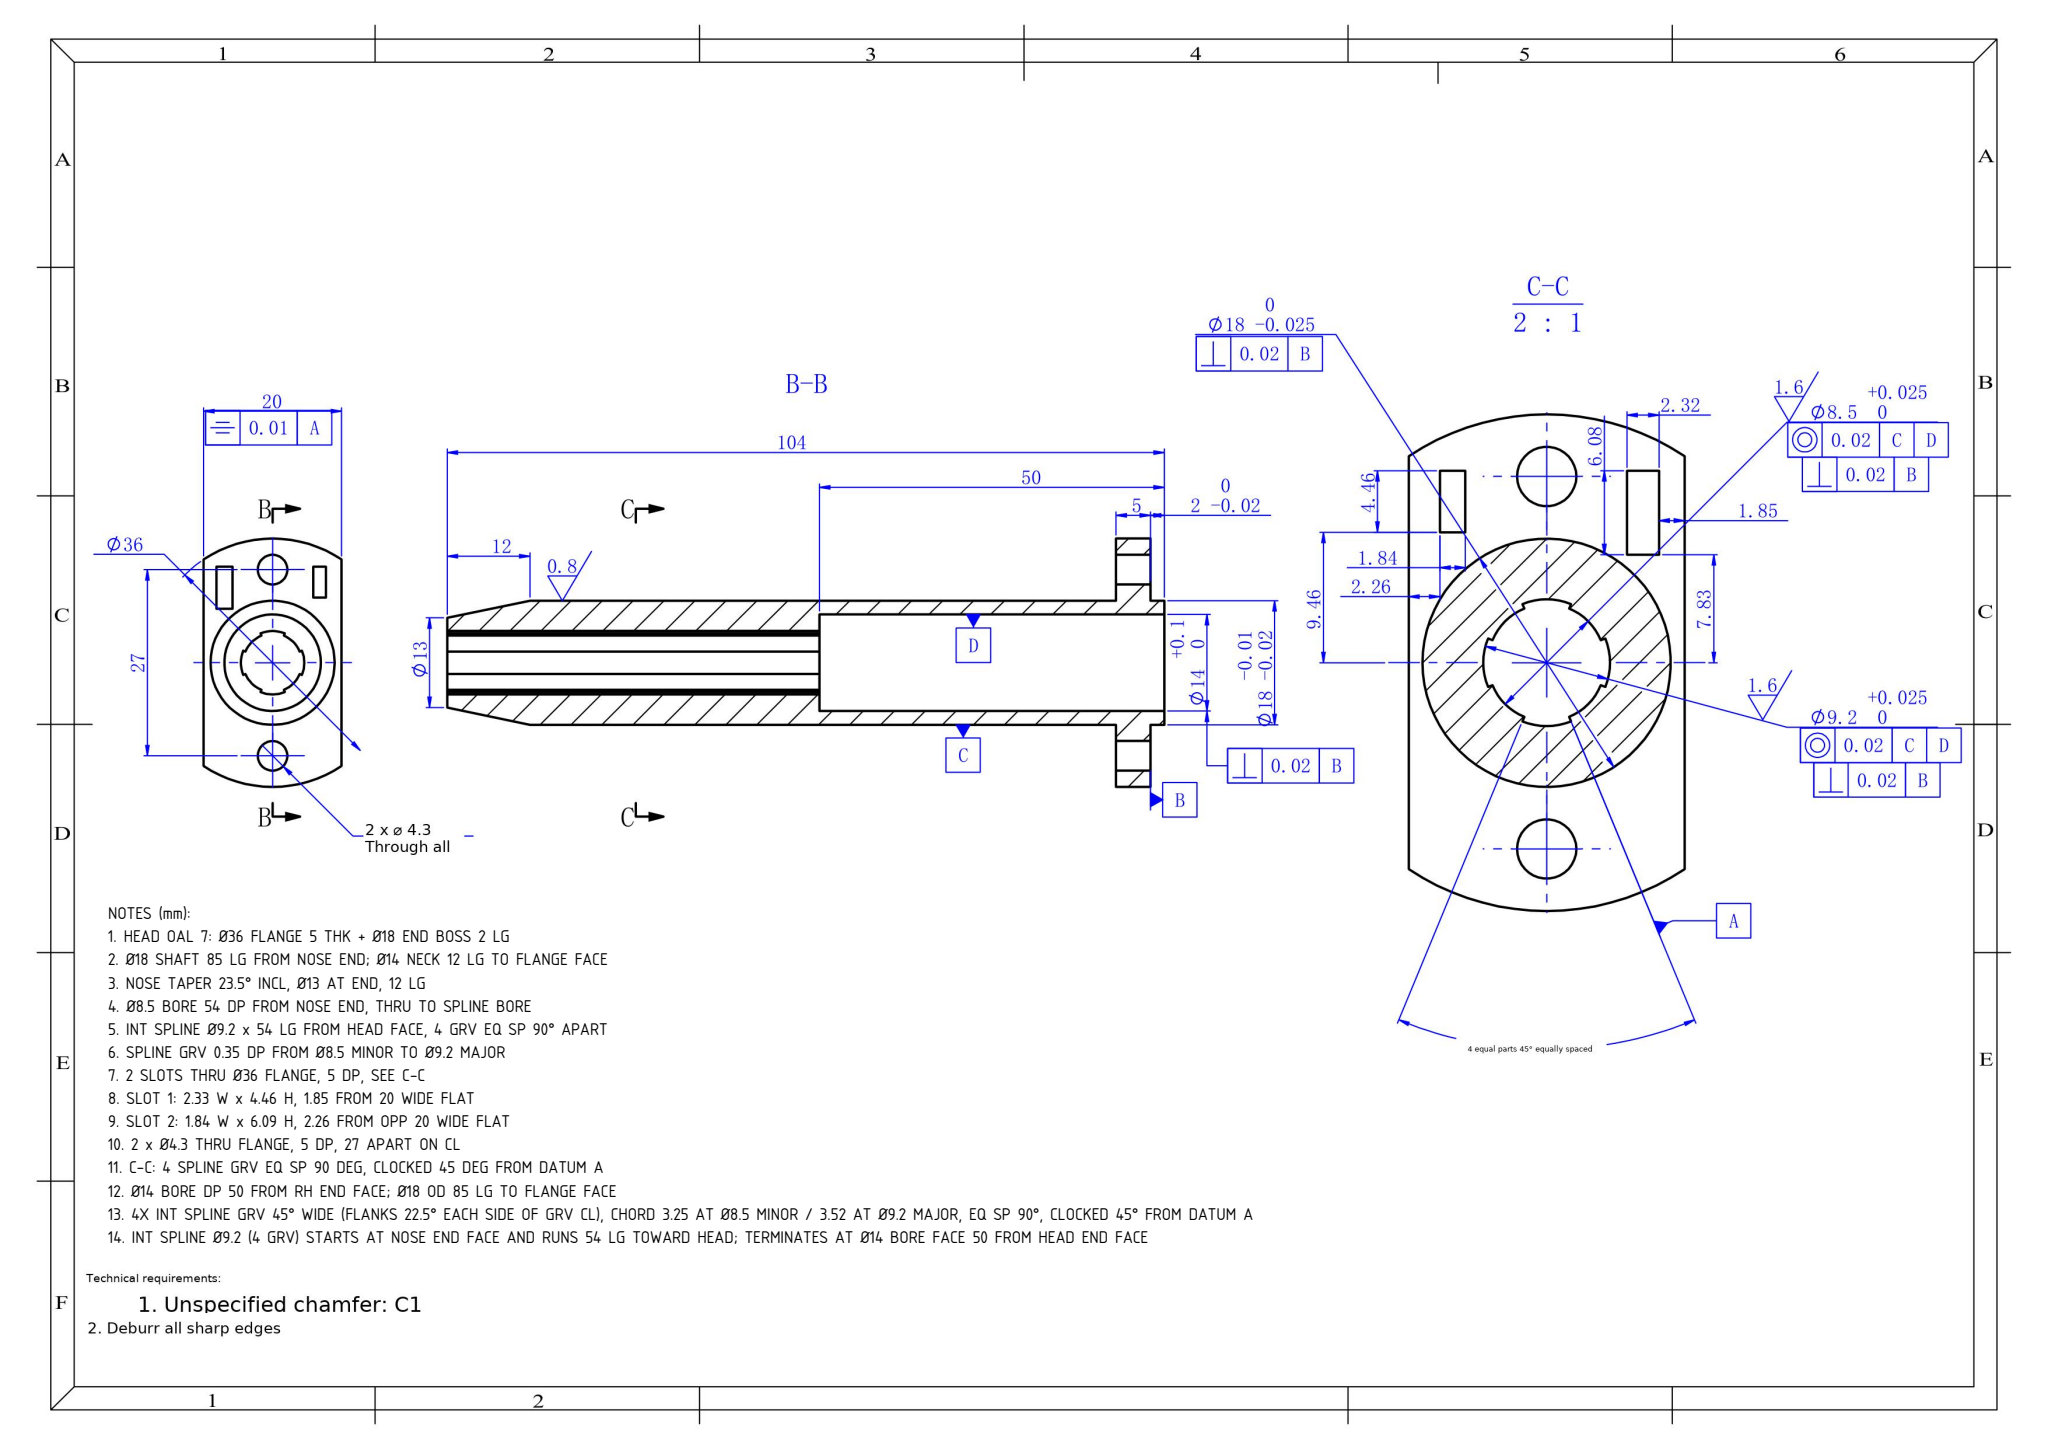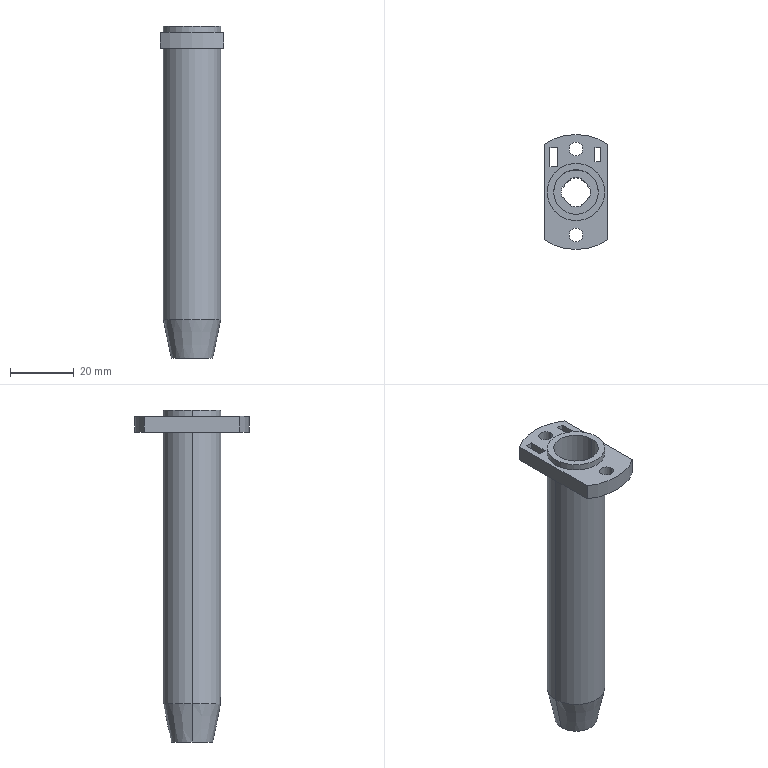Part | SolidWorks | mm | 1 solid | 46 faces | box 20 x 36 x 104 mm | volume 16547 mm3 | plane 23 | cylinder 21 | cone 2 | commonest cylinder face diameters 9.2 x5 18 x4 4.3 x4 8.5 x4 14 x2 36 x2
Drawing notes:
HEAD OAL 7: Ø36 FLANGE 5 THK + Ø18 END BOSS 2 LG | from the solid: Ø36 L=5 (z 97-102) + Ø18 L=2 (z 102-104); z planes 97/102/104
Ø18 SHAFT 85 LG FROM NOSE END; Ø14 NECK 12 LG TO FLANGE FACE | from the solid: Ø18 cyl L=85 (z 0-85); Ø14 cyl z 85-97 = 12
NOSE TAPER 23.5° INCL, Ø13 AT END, 12 LG | from the solid: cones[23.5, ref dia 13]; (18-13)/2/tan11.75°=12
Ø8.5 BORE 54 DP FROM NOSE END, THRU TO SPLINE BORE | from the solid: Ø8.5 cyl L=54 on axis (10,18); bore runs thru 104
INT SPLINE Ø9.2 x 54 LG FROM HEAD FACE, 4 GRV EQ SP 90° APART | from the solid: Ø9.2 cyl L=54 (z 104-50), 4 grooves equally spaced = 90° pitch
SPLINE GRV 0.35 DP FROM Ø8.5 MINOR TO Ø9.2 MAJOR | from the solid: (9.2-8.5)/2 = 0.35
2 SLOTS THRU Ø36 FLANGE, 5 DP, SEE C-C | from the solid: no z planes between 97 and 102; flange thk 5
SLOT 1: 2.33 W x 4.46 H, 1.85 FROM 20 WIDE FLAT | from the solid: x planes 1.85/4.18; y planes 27.46/31.92
SLOT 2: 1.84 W x 6.09 H, 2.26 FROM OPP 20 WIDE FLAT | from the solid: x planes 15.9/17.74; y planes 25.83/31.92
2 x Ø4.3 THRU FLANGE, 5 DP, 27 APART ON CL | from the solid: Ø4.3 cyls L=5 at (10,4.5) and (10,31.5)
C-C: 4 SPLINE GRV EQ SP 90 DEG, CLOCKED 45 DEG FROM DATUM A | from the solid: Bore Ø8.5/Ø9.2 at (10,18); no X- or Y-normal planes exist near bore (only x=0,1.85,4.18,15.9,17.74,20 and y=25.83,27.46,31.92 belonging to the outer pockets), so groove flanks are radial planes not parallel/normal to the 20-wide datum A flats (x=0 / x=20), i.e. grooves lie on the 45 deg bisectors.
Ø14 BORE DP 50 FROM RH END FACE; Ø18 OD 85 LG TO FLANGE FACE | from the solid: cyl Ø14 L=50 and cyl Ø18 L=85 on axis [10,18]; z planes 0/54/97/102/104; 23.5 deg cone ref Ø13 = 12 lg taper at tip, so Ø14 is a 50 deep bore from z=104 end meeting Ø9.2 spline bore at z=54, not a 12 lg neck
4X INT SPLINE GRV 45° WIDE (FLANKS 22.5° EACH SIDE OF GRV CL), CHORD 3.25 AT Ø8.5 MINOR / 3.52 AT Ø9.2 MAJOR, EQ SP 90°, CLOCKED 45° FROM DATUM A | from the solid: 8 inclined_planes (4 grooves x 2 flanks) with normals at 22.5°/67.5° to X/Y, corners at R4.25 (Ø8.5 minor) and R4.60 (Ø9.2 major) about bore axis (10,18), groove CL at 45°
INT SPLINE Ø9.2 (4 GRV) STARTS AT NOSE END FACE AND RUNS 54 LG TOWARD HEAD; TERMINATES AT Ø14 BORE FACE 50 FROM HEAD END FACE | from the solid: cylinders: Ø9.2 and Ø8.5 partial bores z = 0 to 54 (nose end at z0); Ø14 hole/bore z = 54 to 104 (head end face z104); planar face z=54
build123d program:
from build123d import *

# Parameters (mm, degrees)
SKETCH1_R                  = 9
BOSS_EXTRUDE1_DEPTH        = 97
SKETCH2_R                  = 18
BOSS_EXTRUDE2_DEPTH        = 5
SKETCH3_R                  = 4.25
CUT_EXTRUDE1_DEPTH         = 106.128
CUT_EXTRUDE2_DEPTH         = 106.128
SKETCH5_R                  = 7
CUT_EXTRUDE3_DEPTH         = 48
SKETCH6_OUTSIDE_W          = 60.8
SKETCH6_OUTSIDE_H          = 60.8
SKETCH6_OUTSIDE_W_2        = 20
SKETCH6_OUTSIDE_H_2        = 51.011
CUT_EXTRUDE4_DEPTH         = 38
F_4_3_4_3_DIAMETER_HOLE1_D = 4.3
SKETCH13_R                 = 9
SKETCH13_R_2               = 7
BOSS_EXTRUDE3_DEPTH        = 2
SKETCH14_W                 = 1.843
SKETCH14_H                 = 4.461
SKETCH14_W_2               = 2.322
SKETCH14_H_2               = 6.083
CUT_EXTRUDE5_DEPTH         = 10


with BuildPart() as part:
    # Sketch1 → Boss-Extrude1 (new body)
    with BuildSketch(Plane.XY):
        with Locations(Location((0, 0, 0), (0, 0, 180))):
            Circle(SKETCH1_R)
    extrude(amount=BOSS_EXTRUDE1_DEPTH)

    # Sketch2 → Boss-Extrude2 (add)
    with BuildSketch(Plane.XY.offset(97)):
        Circle(SKETCH2_R)
    extrude(amount=BOSS_EXTRUDE2_DEPTH)

    # Sketch3 → Cut-Extrude1 (cut, through all)
    with BuildSketch(Plane(origin=(0, 0, 0), x_dir=(-1, 0, 0), z_dir=(0, 0, -1))):
        Circle(SKETCH3_R)
    extrude(amount=-CUT_EXTRUDE1_DEPTH, mode=Mode.SUBTRACT)

    # Sketch4 → Cut-Extrude2 (cut, through all)
    with BuildSketch(Plane(origin=(0, 0, 0), x_dir=(-1, 0, 0), z_dir=(0, 0, -1))):
        with BuildLine():
            Line((-1.76, 4.25), (-0.8802, 2.125))
            ThreePointArc((-0.8802, 2.125), (0, 2.3), (0.8802, 2.125))
            Line((0.8802, 2.125), (1.76, 4.25))
            ThreePointArc((1.76, 4.25), (0, 4.6), (-1.76, 4.25))
        make_face()
        with BuildLine():
            Line((4.25, -1.76), (2.125, -0.8802))
            ThreePointArc((2.125, -0.8802), (2.3, 0), (2.125, 0.8802))
            Line((2.125, 0.8802), (4.25, 1.76))
            ThreePointArc((4.25, 1.76), (4.6, 0), (4.25, -1.76))
        make_face()
        with BuildLine():
            Line((-1.76, -4.25), (-0.8802, -2.125))
            ThreePointArc((-0.8802, -2.125), (0, -2.3), (0.8802, -2.125))
            Line((0.8802, -2.125), (1.76, -4.25))
            ThreePointArc((1.76, -4.25), (0, -4.6), (-1.76, -4.25))
        make_face()
        with BuildLine():
            Line((-4.25, 1.76), (-2.125, 0.8802))
            ThreePointArc((-2.125, 0.8802), (-2.3, 0), (-2.125, -0.8802))
            Line((-2.125, -0.8802), (-4.25, -1.76))
            ThreePointArc((-4.25, -1.76), (-4.6, 0), (-4.25, 1.76))
        make_face()
    extrude(amount=-CUT_EXTRUDE2_DEPTH, mode=Mode.SUBTRACT)

    # Sketch5 → Cut-Extrude3 (cut)
    with BuildSketch(Plane.XY.offset(102)):
        Circle(SKETCH5_R)
    extrude(amount=-CUT_EXTRUDE3_DEPTH, mode=Mode.SUBTRACT)

    # Sketch6 outside → Cut-Extrude4 (cut)
    with BuildSketch(Plane.XY.offset(102)):
        Rectangle(SKETCH6_OUTSIDE_W, SKETCH6_OUTSIDE_H)
        with Locations((0, -1.305)):
            Rectangle(SKETCH6_OUTSIDE_W_2, SKETCH6_OUTSIDE_H_2, mode=Mode.SUBTRACT)
    extrude(amount=-CUT_EXTRUDE4_DEPTH, mode=Mode.SUBTRACT)

    # Sketch7 → Cut-Revolve1 (revolve, cut)
    with BuildSketch(Plane(origin=(0, 0, 0), x_dir=(1, 0, 0), z_dir=(0, 1, 0)), mode=Mode.PRIVATE) as cut_revolve1_sk:
        Polygon((6.5, 0), (9, -12), (9, 0), align=None)
    revolve(cut_revolve1_sk.sketch.rotate(Axis((0, 0, 0), (0, 0, 1)), 180), axis=Axis((0, 0, 0), (0, 0, 1)), mode=Mode.SUBTRACT)

    # 4.3 _4.3_ Diameter Hole1 (through all)
    with Locations(Plane(origin=(0, 0, 97), x_dir=(-1, 0, 0), z_dir=(0, 0, -1))):
        with Locations((0, -13.5), (0, 13.5)):
            Hole(F_4_3_4_3_DIAMETER_HOLE1_D / 2)

    # Sketch13 → Boss-Extrude3 (add)
    with BuildSketch(Plane.XY.offset(102)):
        with Locations(Location((0, 0, 0), (0, 0, 180))):
            Circle(SKETCH13_R)
        Circle(SKETCH13_R_2, mode=Mode.SUBTRACT)
    extrude(amount=BOSS_EXTRUDE3_DEPTH)

    # Sketch14 → Cut-Extrude5 (cut)
    with BuildSketch(Plane(origin=(0, 0, 97), x_dir=(-1, 0, 0), z_dir=(0, 0, -1))):
        with Locations((-6.82, 11.686)):
            Rectangle(SKETCH14_W, SKETCH14_H)
        with Locations((6.986, 10.875)):
            Rectangle(SKETCH14_W_2, SKETCH14_H_2)
    extrude(amount=-CUT_EXTRUDE5_DEPTH, mode=Mode.SUBTRACT)


solid = part.part